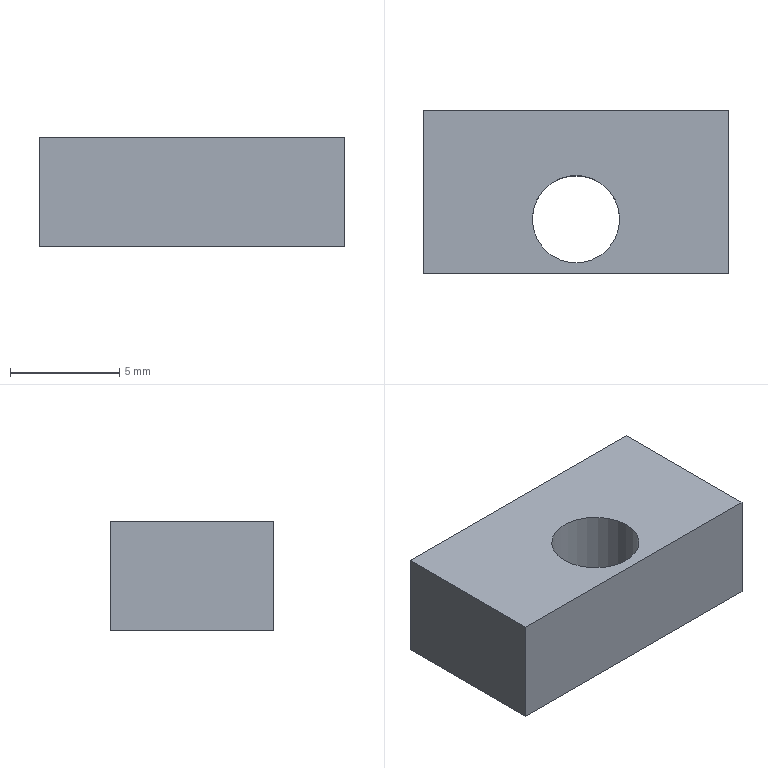Component | NX | SLIDER_BAFFLE | 1 solid | 7 faces | box 14 x 7.5 x 5 mm | volume 462 mm3 | plane 6 | cylinder 1 | commonest cylinder face diameters 4 x1
STEP:
#1=CARTESIAN_POINT('',(0.,0.,0.));
#2=DIRECTION('',(0.,0.,1.));
#3=DIRECTION('',(1.,0.,0.));
#4=AXIS2_PLACEMENT_3D('',#1,#2,#3);
#5=CARTESIAN_POINT('',(7.,20.5,146.131));
#6=VERTEX_POINT('',#5);
#7=CARTESIAN_POINT('',(-7.,20.5,146.131));
#8=VERTEX_POINT('',#7);
#9=CARTESIAN_POINT('',(7.,20.5,146.131));
#10=DIRECTION('',(-1.,0.,0.));
#11=VECTOR('',#10,1.);
#12=LINE('',#9,#11);
#13=CARTESIAN_POINT('',(7.,20.5,141.131));
#14=DIRECTION('',(0.,1.,0.));
#15=DIRECTION('',(0.,0.,-1.));
#16=AXIS2_PLACEMENT_3D('',#13,#14,#15);
#17=PLANE('',#16);
#18=CARTESIAN_POINT('',(-5.,0.));
#19=DIRECTION('',(0.,1.));
#20=VECTOR('',#19,1.);
#21=LINE('',#18,#20);
#22=(GEOMETRIC_REPRESENTATION_CONTEXT(2)PARAMETRIC_REPRESENTATION_CONTEXT()REPRESENTATION_CONTEXT('',''));
#23=DEFINITIONAL_REPRESENTATION('',(#21),#22);
#24=PCURVE('',#17,#23);
#25=CARTESIAN_POINT('',(-0.,23.,146.131));
#26=DIRECTION('',(0.,0.,-1.));
#27=DIRECTION('',(0.,-1.,0.));
#28=AXIS2_PLACEMENT_3D('',#25,#26,#27);
#29=PLANE('',#28);
#30=CARTESIAN_POINT('',(2.5,-7.));
#31=DIRECTION('',(0.,1.));
#32=VECTOR('',#31,1.);
#33=LINE('',#30,#32);
#34=(GEOMETRIC_REPRESENTATION_CONTEXT(2)PARAMETRIC_REPRESENTATION_CONTEXT()REPRESENTATION_CONTEXT('',''));
#35=DEFINITIONAL_REPRESENTATION('',(#33),#34);
#36=PCURVE('',#29,#35);
#37=SURFACE_CURVE('',#12,(#24,#36),.PCURVE_S1.);
#38=EDGE_CURVE('',#6,#8,#37,.T.);
#39=ORIENTED_EDGE('',*,*,#38,.T.);
#40=CARTESIAN_POINT('',(-7.,20.5,141.131));
#41=VERTEX_POINT('',#40);
#42=CARTESIAN_POINT('',(-7.,20.5,141.131));
#43=DIRECTION('',(0.,0.,1.));
#44=VECTOR('',#43,1.);
#45=LINE('',#42,#44);
#46=CARTESIAN_POINT('',(0.,14.));
#47=DIRECTION('',(-1.,0.));
#48=VECTOR('',#47,1.);
#49=LINE('',#46,#48);
#50=(GEOMETRIC_REPRESENTATION_CONTEXT(2)PARAMETRIC_REPRESENTATION_CONTEXT()REPRESENTATION_CONTEXT('',''));
#51=DEFINITIONAL_REPRESENTATION('',(#49),#50);
#52=PCURVE('',#17,#51);
#53=CARTESIAN_POINT('',(-7.,20.5,141.131));
#54=DIRECTION('',(1.,0.,0.));
#55=DIRECTION('',(0.,-1.,0.));
#56=AXIS2_PLACEMENT_3D('',#53,#54,#55);
#57=PLANE('',#56);
#58=CARTESIAN_POINT('',(0.,0.));
#59=DIRECTION('',(0.,-1.));
#60=VECTOR('',#59,1.);
#61=LINE('',#58,#60);
#62=(GEOMETRIC_REPRESENTATION_CONTEXT(2)PARAMETRIC_REPRESENTATION_CONTEXT()REPRESENTATION_CONTEXT('',''));
#63=DEFINITIONAL_REPRESENTATION('',(#61),#62);
#64=PCURVE('',#57,#63);
#65=SURFACE_CURVE('',#45,(#52,#64),.PCURVE_S1.);
#66=EDGE_CURVE('',#41,#8,#65,.T.);
#67=ORIENTED_EDGE('',*,*,#66,.F.);
#68=CARTESIAN_POINT('',(7.,20.5,141.131));
#69=VERTEX_POINT('',#68);
#70=CARTESIAN_POINT('',(7.,20.5,141.131));
#71=DIRECTION('',(-1.,0.,0.));
#72=VECTOR('',#71,1.);
#73=LINE('',#70,#72);
#74=CARTESIAN_POINT('',(0.,0.));
#75=DIRECTION('',(0.,1.));
#76=VECTOR('',#75,1.);
#77=LINE('',#74,#76);
#78=(GEOMETRIC_REPRESENTATION_CONTEXT(2)PARAMETRIC_REPRESENTATION_CONTEXT()REPRESENTATION_CONTEXT('',''));
#79=DEFINITIONAL_REPRESENTATION('',(#77),#78);
#80=PCURVE('',#17,#79);
#81=CARTESIAN_POINT('',(-0.,23.,141.131));
#82=DIRECTION('',(0.,0.,-1.));
#83=DIRECTION('',(0.,-1.,0.));
#84=AXIS2_PLACEMENT_3D('',#81,#82,#83);
#85=PLANE('',#84);
#86=CARTESIAN_POINT('',(2.5,-7.));
#87=DIRECTION('',(0.,1.));
#88=VECTOR('',#87,1.);
#89=LINE('',#86,#88);
#90=(GEOMETRIC_REPRESENTATION_CONTEXT(2)PARAMETRIC_REPRESENTATION_CONTEXT()REPRESENTATION_CONTEXT('',''));
#91=DEFINITIONAL_REPRESENTATION('',(#89),#90);
#92=PCURVE('',#85,#91);
#93=SURFACE_CURVE('',#73,(#80,#92),.PCURVE_S1.);
#94=EDGE_CURVE('',#69,#41,#93,.T.);
#95=ORIENTED_EDGE('',*,*,#94,.F.);
#96=CARTESIAN_POINT('',(7.,20.5,141.131));
#97=DIRECTION('',(0.,0.,1.));
#98=VECTOR('',#97,1.);
#99=LINE('',#96,#98);
#100=CARTESIAN_POINT('',(0.,0.));
#101=DIRECTION('',(-1.,0.));
#102=VECTOR('',#101,1.);
#103=LINE('',#100,#102);
#104=(GEOMETRIC_REPRESENTATION_CONTEXT(2)PARAMETRIC_REPRESENTATION_CONTEXT()REPRESENTATION_CONTEXT('',''));
#105=DEFINITIONAL_REPRESENTATION('',(#103),#104);
#106=PCURVE('',#17,#105);
#107=CARTESIAN_POINT('',(7.,28.,141.131));
#108=DIRECTION('',(-1.,0.,0.));
#109=DIRECTION('',(0.,1.,0.));
#110=AXIS2_PLACEMENT_3D('',#107,#108,#109);
#111=PLANE('',#110);
#112=CARTESIAN_POINT('',(-7.5,0.));
#113=DIRECTION('',(0.,-1.));
#114=VECTOR('',#113,1.);
#115=LINE('',#112,#114);
#116=(GEOMETRIC_REPRESENTATION_CONTEXT(2)PARAMETRIC_REPRESENTATION_CONTEXT()REPRESENTATION_CONTEXT('',''));
#117=DEFINITIONAL_REPRESENTATION('',(#115),#116);
#118=PCURVE('',#111,#117);
#119=SURFACE_CURVE('',#99,(#106,#118),.PCURVE_S1.);
#120=EDGE_CURVE('',#69,#6,#119,.T.);
#121=ORIENTED_EDGE('',*,*,#120,.T.);
#122=EDGE_LOOP('',(#39,#67,#95,#121));
#123=FACE_BOUND('',#122,.T.);
#124=ADVANCED_FACE('',(#123),#17,.F.);
#125=CARTESIAN_POINT('',(-7.,28.,146.131));
#126=VERTEX_POINT('',#125);
#127=CARTESIAN_POINT('',(-7.,20.5,146.131));
#128=DIRECTION('',(0.,1.,0.));
#129=VECTOR('',#128,1.);
#130=LINE('',#127,#129);
#131=CARTESIAN_POINT('',(0.,-5.));
#132=DIRECTION('',(-1.,0.));
#133=VECTOR('',#132,1.);
#134=LINE('',#131,#133);
#135=(GEOMETRIC_REPRESENTATION_CONTEXT(2)PARAMETRIC_REPRESENTATION_CONTEXT()REPRESENTATION_CONTEXT('',''));
#136=DEFINITIONAL_REPRESENTATION('',(#134),#135);
#137=PCURVE('',#57,#136);
#138=CARTESIAN_POINT('',(2.5,7.));
#139=DIRECTION('',(-1.,0.));
#140=VECTOR('',#139,1.);
#141=LINE('',#138,#140);
#142=(GEOMETRIC_REPRESENTATION_CONTEXT(2)PARAMETRIC_REPRESENTATION_CONTEXT()REPRESENTATION_CONTEXT('',''));
#143=DEFINITIONAL_REPRESENTATION('',(#141),#142);
#144=PCURVE('',#29,#143);
#145=SURFACE_CURVE('',#130,(#137,#144),.PCURVE_S1.);
#146=EDGE_CURVE('',#8,#126,#145,.T.);
#147=ORIENTED_EDGE('',*,*,#146,.T.);
#148=CARTESIAN_POINT('',(-7.,28.,141.131));
#149=VERTEX_POINT('',#148);
#150=CARTESIAN_POINT('',(-7.,28.,141.131));
#151=DIRECTION('',(0.,0.,1.));
#152=VECTOR('',#151,1.);
#153=LINE('',#150,#152);
#154=CARTESIAN_POINT('',(-7.5,0.));
#155=DIRECTION('',(0.,-1.));
#156=VECTOR('',#155,1.);
#157=LINE('',#154,#156);
#158=(GEOMETRIC_REPRESENTATION_CONTEXT(2)PARAMETRIC_REPRESENTATION_CONTEXT()REPRESENTATION_CONTEXT('',''));
#159=DEFINITIONAL_REPRESENTATION('',(#157),#158);
#160=PCURVE('',#57,#159);
#161=CARTESIAN_POINT('',(-7.,28.,141.131));
#162=DIRECTION('',(0.,-1.,0.));
#163=DIRECTION('',(0.,0.,1.));
#164=AXIS2_PLACEMENT_3D('',#161,#162,#163);
#165=PLANE('',#164);
#166=CARTESIAN_POINT('',(0.,0.));
#167=DIRECTION('',(1.,0.));
#168=VECTOR('',#167,1.);
#169=LINE('',#166,#168);
#170=(GEOMETRIC_REPRESENTATION_CONTEXT(2)PARAMETRIC_REPRESENTATION_CONTEXT()REPRESENTATION_CONTEXT('',''));
#171=DEFINITIONAL_REPRESENTATION('',(#169),#170);
#172=PCURVE('',#165,#171);
#173=SURFACE_CURVE('',#153,(#160,#172),.PCURVE_S1.);
#174=EDGE_CURVE('',#149,#126,#173,.T.);
#175=ORIENTED_EDGE('',*,*,#174,.F.);
#176=CARTESIAN_POINT('',(-7.,20.5,141.131));
#177=DIRECTION('',(0.,1.,0.));
#178=VECTOR('',#177,1.);
#179=LINE('',#176,#178);
#180=CARTESIAN_POINT('',(0.,0.));
#181=DIRECTION('',(-1.,0.));
#182=VECTOR('',#181,1.);
#183=LINE('',#180,#182);
#184=(GEOMETRIC_REPRESENTATION_CONTEXT(2)PARAMETRIC_REPRESENTATION_CONTEXT()REPRESENTATION_CONTEXT('',''));
#185=DEFINITIONAL_REPRESENTATION('',(#183),#184);
#186=PCURVE('',#57,#185);
#187=CARTESIAN_POINT('',(2.5,7.));
#188=DIRECTION('',(-1.,0.));
#189=VECTOR('',#188,1.);
#190=LINE('',#187,#189);
#191=(GEOMETRIC_REPRESENTATION_CONTEXT(2)PARAMETRIC_REPRESENTATION_CONTEXT()REPRESENTATION_CONTEXT('',''));
#192=DEFINITIONAL_REPRESENTATION('',(#190),#191);
#193=PCURVE('',#85,#192);
#194=SURFACE_CURVE('',#179,(#186,#193),.PCURVE_S1.);
#195=EDGE_CURVE('',#41,#149,#194,.T.);
#196=ORIENTED_EDGE('',*,*,#195,.F.);
#197=ORIENTED_EDGE('',*,*,#66,.T.);
#198=EDGE_LOOP('',(#147,#175,#196,#197));
#199=FACE_BOUND('',#198,.T.);
#200=ADVANCED_FACE('',(#199),#57,.F.);
#201=CARTESIAN_POINT('',(7.,28.,146.131));
#202=VERTEX_POINT('',#201);
#203=CARTESIAN_POINT('',(-7.,28.,146.131));
#204=DIRECTION('',(1.,0.,0.));
#205=VECTOR('',#204,1.);
#206=LINE('',#203,#205);
#207=CARTESIAN_POINT('',(5.,0.));
#208=DIRECTION('',(0.,-1.));
#209=VECTOR('',#208,1.);
#210=LINE('',#207,#209);
#211=(GEOMETRIC_REPRESENTATION_CONTEXT(2)PARAMETRIC_REPRESENTATION_CONTEXT()REPRESENTATION_CONTEXT('',''));
#212=DEFINITIONAL_REPRESENTATION('',(#210),#211);
#213=PCURVE('',#165,#212);
#214=CARTESIAN_POINT('',(-5.,7.));
#215=DIRECTION('',(0.,-1.));
#216=VECTOR('',#215,1.);
#217=LINE('',#214,#216);
#218=(GEOMETRIC_REPRESENTATION_CONTEXT(2)PARAMETRIC_REPRESENTATION_CONTEXT()REPRESENTATION_CONTEXT('',''));
#219=DEFINITIONAL_REPRESENTATION('',(#217),#218);
#220=PCURVE('',#29,#219);
#221=SURFACE_CURVE('',#206,(#213,#220),.PCURVE_S1.);
#222=EDGE_CURVE('',#126,#202,#221,.T.);
#223=ORIENTED_EDGE('',*,*,#222,.T.);
#224=CARTESIAN_POINT('',(7.,28.,141.131));
#225=VERTEX_POINT('',#224);
#226=CARTESIAN_POINT('',(7.,28.,141.131));
#227=DIRECTION('',(0.,0.,1.));
#228=VECTOR('',#227,1.);
#229=LINE('',#226,#228);
#230=CARTESIAN_POINT('',(0.,-14.));
#231=DIRECTION('',(1.,0.));
#232=VECTOR('',#231,1.);
#233=LINE('',#230,#232);
#234=(GEOMETRIC_REPRESENTATION_CONTEXT(2)PARAMETRIC_REPRESENTATION_CONTEXT()REPRESENTATION_CONTEXT('',''));
#235=DEFINITIONAL_REPRESENTATION('',(#233),#234);
#236=PCURVE('',#165,#235);
#237=CARTESIAN_POINT('',(0.,0.));
#238=DIRECTION('',(0.,-1.));
#239=VECTOR('',#238,1.);
#240=LINE('',#237,#239);
#241=(GEOMETRIC_REPRESENTATION_CONTEXT(2)PARAMETRIC_REPRESENTATION_CONTEXT()REPRESENTATION_CONTEXT('',''));
#242=DEFINITIONAL_REPRESENTATION('',(#240),#241);
#243=PCURVE('',#111,#242);
#244=SURFACE_CURVE('',#229,(#236,#243),.PCURVE_S1.);
#245=EDGE_CURVE('',#225,#202,#244,.T.);
#246=ORIENTED_EDGE('',*,*,#245,.F.);
#247=CARTESIAN_POINT('',(-7.,28.,141.131));
#248=DIRECTION('',(1.,0.,0.));
#249=VECTOR('',#248,1.);
#250=LINE('',#247,#249);
#251=CARTESIAN_POINT('',(0.,0.));
#252=DIRECTION('',(0.,-1.));
#253=VECTOR('',#252,1.);
#254=LINE('',#251,#253);
#255=(GEOMETRIC_REPRESENTATION_CONTEXT(2)PARAMETRIC_REPRESENTATION_CONTEXT()REPRESENTATION_CONTEXT('',''));
#256=DEFINITIONAL_REPRESENTATION('',(#254),#255);
#257=PCURVE('',#165,#256);
#258=CARTESIAN_POINT('',(-5.,7.));
#259=DIRECTION('',(0.,-1.));
#260=VECTOR('',#259,1.);
#261=LINE('',#258,#260);
#262=(GEOMETRIC_REPRESENTATION_CONTEXT(2)PARAMETRIC_REPRESENTATION_CONTEXT()REPRESENTATION_CONTEXT('',''));
#263=DEFINITIONAL_REPRESENTATION('',(#261),#262);
#264=PCURVE('',#85,#263);
#265=SURFACE_CURVE('',#250,(#257,#264),.PCURVE_S1.);
#266=EDGE_CURVE('',#149,#225,#265,.T.);
#267=ORIENTED_EDGE('',*,*,#266,.F.);
#268=ORIENTED_EDGE('',*,*,#174,.T.);
#269=EDGE_LOOP('',(#223,#246,#267,#268));
#270=FACE_BOUND('',#269,.T.);
#271=ADVANCED_FACE('',(#270),#165,.F.);
#272=CARTESIAN_POINT('',(7.,28.,146.131));
#273=DIRECTION('',(0.,-1.,0.));
#274=VECTOR('',#273,1.);
#275=LINE('',#272,#274);
#276=CARTESIAN_POINT('',(0.,-5.));
#277=DIRECTION('',(-1.,0.));
#278=VECTOR('',#277,1.);
#279=LINE('',#276,#278);
#280=(GEOMETRIC_REPRESENTATION_CONTEXT(2)PARAMETRIC_REPRESENTATION_CONTEXT()REPRESENTATION_CONTEXT('',''));
#281=DEFINITIONAL_REPRESENTATION('',(#279),#280);
#282=PCURVE('',#111,#281);
#283=CARTESIAN_POINT('',(-5.,-7.));
#284=DIRECTION('',(1.,0.));
#285=VECTOR('',#284,1.);
#286=LINE('',#283,#285);
#287=(GEOMETRIC_REPRESENTATION_CONTEXT(2)PARAMETRIC_REPRESENTATION_CONTEXT()REPRESENTATION_CONTEXT('',''));
#288=DEFINITIONAL_REPRESENTATION('',(#286),#287);
#289=PCURVE('',#29,#288);
#290=SURFACE_CURVE('',#275,(#282,#289),.PCURVE_S1.);
#291=EDGE_CURVE('',#202,#6,#290,.T.);
#292=ORIENTED_EDGE('',*,*,#291,.T.);
#293=ORIENTED_EDGE('',*,*,#120,.F.);
#294=CARTESIAN_POINT('',(7.,28.,141.131));
#295=DIRECTION('',(0.,-1.,0.));
#296=VECTOR('',#295,1.);
#297=LINE('',#294,#296);
#298=CARTESIAN_POINT('',(0.,0.));
#299=DIRECTION('',(-1.,0.));
#300=VECTOR('',#299,1.);
#301=LINE('',#298,#300);
#302=(GEOMETRIC_REPRESENTATION_CONTEXT(2)PARAMETRIC_REPRESENTATION_CONTEXT()REPRESENTATION_CONTEXT('',''));
#303=DEFINITIONAL_REPRESENTATION('',(#301),#302);
#304=PCURVE('',#111,#303);
#305=CARTESIAN_POINT('',(-5.,-7.));
#306=DIRECTION('',(1.,0.));
#307=VECTOR('',#306,1.);
#308=LINE('',#305,#307);
#309=(GEOMETRIC_REPRESENTATION_CONTEXT(2)PARAMETRIC_REPRESENTATION_CONTEXT()REPRESENTATION_CONTEXT('',''));
#310=DEFINITIONAL_REPRESENTATION('',(#308),#309);
#311=PCURVE('',#85,#310);
#312=SURFACE_CURVE('',#297,(#304,#311),.PCURVE_S1.);
#313=EDGE_CURVE('',#225,#69,#312,.T.);
#314=ORIENTED_EDGE('',*,*,#313,.F.);
#315=ORIENTED_EDGE('',*,*,#245,.T.);
#316=EDGE_LOOP('',(#292,#293,#314,#315));
#317=FACE_BOUND('',#316,.T.);
#318=ADVANCED_FACE('',(#317),#111,.F.);
#319=CARTESIAN_POINT('',(-2.,23.,141.131));
#320=VERTEX_POINT('',#319);
#321=CARTESIAN_POINT('',(-0.,23.,141.131));
#322=DIRECTION('',(0.,0.,-1.));
#323=DIRECTION('',(-1.,0.,0.));
#324=AXIS2_PLACEMENT_3D('',#321,#322,#323);
#325=CIRCLE('',#324,2.);
#326=CARTESIAN_POINT('',(-0.,23.,141.131));
#327=DIRECTION('',(0.,0.,1.));
#328=DIRECTION('',(0.,1.,0.));
#329=AXIS2_PLACEMENT_3D('',#326,#327,#328);
#330=CYLINDRICAL_SURFACE('',#329,2.);
#331=CARTESIAN_POINT('',(7.854,0.));
#332=DIRECTION('',(-1.,0.));
#333=VECTOR('',#332,1.);
#334=LINE('',#331,#333);
#335=(GEOMETRIC_REPRESENTATION_CONTEXT(2)PARAMETRIC_REPRESENTATION_CONTEXT()REPRESENTATION_CONTEXT('',''));
#336=DEFINITIONAL_REPRESENTATION('',(#334),#335);
#337=PCURVE('',#330,#336);
#338=CARTESIAN_POINT('',(0.,0.));
#339=DIRECTION('',(0.,1.));
#340=AXIS2_PLACEMENT_2D('',#338,#339);
#341=CIRCLE('',#340,2.);
#342=(GEOMETRIC_REPRESENTATION_CONTEXT(2)PARAMETRIC_REPRESENTATION_CONTEXT()REPRESENTATION_CONTEXT('',''));
#343=DEFINITIONAL_REPRESENTATION('',(#341),#342);
#344=PCURVE('',#85,#343);
#345=SURFACE_CURVE('',#325,(#337,#344),.PCURVE_S1.);
#346=EDGE_CURVE('',#320,#320,#345,.T.);
#347=ORIENTED_EDGE('',*,*,#346,.F.);
#348=CARTESIAN_POINT('',(-2.,23.,146.131));
#349=VERTEX_POINT('',#348);
#350=CARTESIAN_POINT('',(-2.,23.,141.131));
#351=CARTESIAN_POINT('',(-2.,23.,146.131));
#352=B_SPLINE_CURVE_WITH_KNOTS('',1,(#350,#351),.UNSPECIFIED.,.F.,.F.,(2,2),(0.,5.),.PIECEWISE_BEZIER_KNOTS.);
#353=CARTESIAN_POINT('',(7.854,0.));
#354=DIRECTION('',(0.,1.));
#355=VECTOR('',#354,1.);
#356=LINE('',#353,#355);
#357=(GEOMETRIC_REPRESENTATION_CONTEXT(2)PARAMETRIC_REPRESENTATION_CONTEXT()REPRESENTATION_CONTEXT('',''));
#358=DEFINITIONAL_REPRESENTATION('',(#356),#357);
#359=PCURVE('',#330,#358);
#360=CARTESIAN_POINT('',(1.571,0.));
#361=DIRECTION('',(0.,1.));
#362=VECTOR('',#361,1.);
#363=LINE('',#360,#362);
#364=(GEOMETRIC_REPRESENTATION_CONTEXT(2)PARAMETRIC_REPRESENTATION_CONTEXT()REPRESENTATION_CONTEXT('',''));
#365=DEFINITIONAL_REPRESENTATION('',(#363),#364);
#366=PCURVE('',#330,#365);
#367=SEAM_CURVE('',#352,(#359,#366),.PCURVE_S1.);
#368=EDGE_CURVE('',#320,#349,#367,.T.);
#369=ORIENTED_EDGE('',*,*,#368,.T.);
#370=CARTESIAN_POINT('',(-0.,23.,146.131));
#371=DIRECTION('',(0.,0.,-1.));
#372=DIRECTION('',(-1.,0.,0.));
#373=AXIS2_PLACEMENT_3D('',#370,#371,#372);
#374=CIRCLE('',#373,2.);
#375=CARTESIAN_POINT('',(7.854,5.));
#376=DIRECTION('',(-1.,0.));
#377=VECTOR('',#376,1.);
#378=LINE('',#375,#377);
#379=(GEOMETRIC_REPRESENTATION_CONTEXT(2)PARAMETRIC_REPRESENTATION_CONTEXT()REPRESENTATION_CONTEXT('',''));
#380=DEFINITIONAL_REPRESENTATION('',(#378),#379);
#381=PCURVE('',#330,#380);
#382=CARTESIAN_POINT('',(0.,0.));
#383=DIRECTION('',(0.,1.));
#384=AXIS2_PLACEMENT_2D('',#382,#383);
#385=CIRCLE('',#384,2.);
#386=(GEOMETRIC_REPRESENTATION_CONTEXT(2)PARAMETRIC_REPRESENTATION_CONTEXT()REPRESENTATION_CONTEXT('',''));
#387=DEFINITIONAL_REPRESENTATION('',(#385),#386);
#388=PCURVE('',#29,#387);
#389=SURFACE_CURVE('',#374,(#381,#388),.PCURVE_S1.);
#390=EDGE_CURVE('',#349,#349,#389,.T.);
#391=ORIENTED_EDGE('',*,*,#390,.T.);
#392=ORIENTED_EDGE('',*,*,#368,.F.);
#393=EDGE_LOOP('',(#347,#369,#391,#392));
#394=FACE_BOUND('',#393,.F.);
#395=ADVANCED_FACE('',(#394),#330,.F.);
#396=ORIENTED_EDGE('',*,*,#94,.T.);
#397=ORIENTED_EDGE('',*,*,#195,.T.);
#398=ORIENTED_EDGE('',*,*,#266,.T.);
#399=ORIENTED_EDGE('',*,*,#313,.T.);
#400=EDGE_LOOP('',(#396,#397,#398,#399));
#401=FACE_BOUND('',#400,.T.);
#402=ORIENTED_EDGE('',*,*,#346,.F.);
#403=EDGE_LOOP('',(#402));
#404=FACE_BOUND('',#403,.T.);
#405=ADVANCED_FACE('',(#401,#404),#85,.T.);
#406=ORIENTED_EDGE('',*,*,#38,.F.);
#407=ORIENTED_EDGE('',*,*,#291,.F.);
#408=ORIENTED_EDGE('',*,*,#222,.F.);
#409=ORIENTED_EDGE('',*,*,#146,.F.);
#410=EDGE_LOOP('',(#406,#407,#408,#409));
#411=FACE_BOUND('',#410,.T.);
#412=ORIENTED_EDGE('',*,*,#390,.T.);
#413=EDGE_LOOP('',(#412));
#414=FACE_BOUND('',#413,.T.);
#415=ADVANCED_FACE('',(#411,#414),#29,.F.);
#416=CLOSED_SHELL('',(#124,#200,#271,#318,#395,#405,#415));
#417=MANIFOLD_SOLID_BREP('',#416);
#418=(LENGTH_UNIT()NAMED_UNIT(*)SI_UNIT(.MILLI.,.METRE.));
#419=UNCERTAINTY_MEASURE_WITH_UNIT(LENGTH_MEASURE(0.000002),#418,'','');
#420=(NAMED_UNIT(*)PLANE_ANGLE_UNIT()SI_UNIT($,.RADIAN.));
#421=(NAMED_UNIT(*)SI_UNIT($,.STERADIAN.)SOLID_ANGLE_UNIT());
#422=(GEOMETRIC_REPRESENTATION_CONTEXT(3)GLOBAL_UNCERTAINTY_ASSIGNED_CONTEXT((#419))GLOBAL_UNIT_ASSIGNED_CONTEXT((#418,#420,#421))REPRESENTATION_CONTEXT('',''));
#423=ADVANCED_BREP_SHAPE_REPRESENTATION('',(#4,#417),#422);